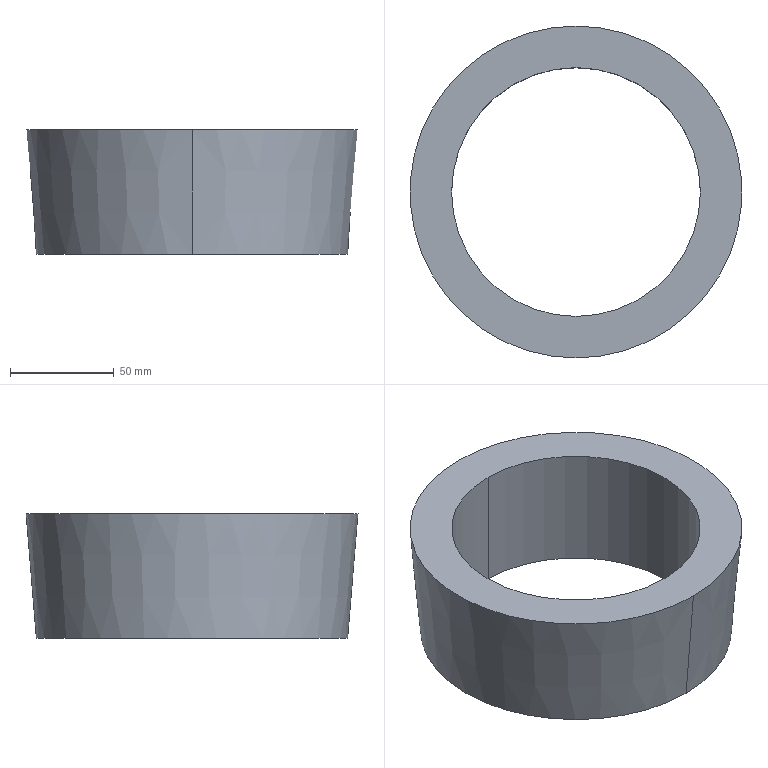Component | SolidWorks | DieCore-1 | 1 solid | 6 faces | box 160.14 x 160.14 x 60 mm | volume 455986 mm3 | cylinder 2 | cone 2 | plane 2 | commonest cylinder face diameters 120 x2
STEP:
#1=CARTESIAN_POINT('',(0.,-2.362,-1.89));
#2=VERTEX_POINT('',#1);
#3=CARTESIAN_POINT('',(-0.,2.362,-1.89));
#4=VERTEX_POINT('',#3);
#5=CARTESIAN_POINT('',(0.,-0.,-1.89));
#6=DIRECTION('',(-0.,0.,-1.));
#7=DIRECTION('',(0.,-1.,-0.));
#8=AXIS2_PLACEMENT_3D('',#5,#6,#7);
#9=CIRCLE('',#8,2.362);
#10=EDGE_CURVE('',#2,#4,#9,.T.);
#11=ORIENTED_EDGE('',*,*,#10,.F.);
#12=CARTESIAN_POINT('',(0.,-2.362,-4.252));
#13=VERTEX_POINT('',#12);
#14=CARTESIAN_POINT('',(0.,-2.362,3.94));
#15=DIRECTION('',(-0.,0.,-1.));
#16=VECTOR('',#15,39.37);
#17=LINE('',#14,#16);
#18=EDGE_CURVE('',#2,#13,#17,.T.);
#19=ORIENTED_EDGE('',*,*,#18,.T.);
#20=CARTESIAN_POINT('',(-0.,2.362,-4.252));
#21=VERTEX_POINT('',#20);
#22=CARTESIAN_POINT('',(0.,-0.,-4.252));
#23=DIRECTION('',(-0.,0.,-1.));
#24=DIRECTION('',(-0.,1.,0.));
#25=AXIS2_PLACEMENT_3D('',#22,#23,#24);
#26=CIRCLE('',#25,2.362);
#27=EDGE_CURVE('',#13,#21,#26,.T.);
#28=ORIENTED_EDGE('',*,*,#27,.T.);
#29=CARTESIAN_POINT('',(0.,2.362,3.94));
#30=DIRECTION('',(-0.,0.,-1.));
#31=VECTOR('',#30,39.37);
#32=LINE('',#29,#31);
#33=EDGE_CURVE('',#4,#21,#32,.T.);
#34=ORIENTED_EDGE('',*,*,#33,.F.);
#35=EDGE_LOOP('',(#11,#19,#28,#34));
#36=FACE_OUTER_BOUND('',#35,.T.);
#37=CARTESIAN_POINT('',(0.,-0.,3.94));
#38=DIRECTION('',(-0.,0.,-1.));
#39=DIRECTION('',(-0.,1.,0.));
#40=AXIS2_PLACEMENT_3D('',#37,#38,#39);
#41=CYLINDRICAL_SURFACE('',#40,2.362);
#42=ADVANCED_FACE('',(#36),#41,.F.);
#43=CARTESIAN_POINT('',(0.,2.955,-4.252));
#44=VERTEX_POINT('',#43);
#45=CARTESIAN_POINT('',(0.,-2.955,-4.252));
#46=VERTEX_POINT('',#45);
#47=CARTESIAN_POINT('',(0.,-0.,-4.252));
#48=DIRECTION('',(-0.,0.,-1.));
#49=DIRECTION('',(-0.,1.,0.));
#50=AXIS2_PLACEMENT_3D('',#47,#48,#49);
#51=CIRCLE('',#50,2.955);
#52=EDGE_CURVE('',#44,#46,#51,.T.);
#53=ORIENTED_EDGE('',*,*,#52,.F.);
#54=CARTESIAN_POINT('',(0.,3.152,-1.89));
#55=VERTEX_POINT('',#54);
#56=CARTESIAN_POINT('',(-0.,2.95,-4.317));
#57=DIRECTION('',(0.,0.08305,0.9965));
#58=VECTOR('',#57,39.37);
#59=LINE('',#56,#58);
#60=EDGE_CURVE('',#44,#55,#59,.T.);
#61=ORIENTED_EDGE('',*,*,#60,.T.);
#62=CARTESIAN_POINT('',(0.,-3.152,-1.89));
#63=VERTEX_POINT('',#62);
#64=CARTESIAN_POINT('',(0.,-0.,-1.89));
#65=DIRECTION('',(-0.,0.,-1.));
#66=DIRECTION('',(0.,-1.,-0.));
#67=AXIS2_PLACEMENT_3D('',#64,#65,#66);
#68=CIRCLE('',#67,3.152);
#69=EDGE_CURVE('',#55,#63,#68,.T.);
#70=ORIENTED_EDGE('',*,*,#69,.T.);
#71=CARTESIAN_POINT('',(0.,-2.95,-4.317));
#72=DIRECTION('',(0.,-0.08305,0.9965));
#73=VECTOR('',#72,39.37);
#74=LINE('',#71,#73);
#75=EDGE_CURVE('',#46,#63,#74,.T.);
#76=ORIENTED_EDGE('',*,*,#75,.F.);
#77=EDGE_LOOP('',(#53,#61,#70,#76));
#78=FACE_OUTER_BOUND('',#77,.T.);
#79=CARTESIAN_POINT('',(0.,-0.,-4.317));
#80=DIRECTION('',(0.,-0.,1.));
#81=DIRECTION('',(0.,-1.,-0.));
#82=AXIS2_PLACEMENT_3D('',#79,#80,#81);
#83=CONICAL_SURFACE('',#82,2.95,0.08314);
#84=ADVANCED_FACE('',(#78),#83,.T.);
#85=CARTESIAN_POINT('',(0.,-0.,-1.89));
#86=DIRECTION('',(-0.,0.,-1.));
#87=DIRECTION('',(0.,-1.,-0.));
#88=AXIS2_PLACEMENT_3D('',#85,#86,#87);
#89=CIRCLE('',#88,3.152);
#90=EDGE_CURVE('',#63,#55,#89,.T.);
#91=ORIENTED_EDGE('',*,*,#90,.F.);
#92=ORIENTED_EDGE('',*,*,#69,.F.);
#93=EDGE_LOOP('',(#91,#92));
#94=FACE_OUTER_BOUND('',#93,.T.);
#95=CARTESIAN_POINT('',(0.,-0.,-1.89));
#96=DIRECTION('',(-0.,0.,-1.));
#97=DIRECTION('',(0.,-1.,-0.));
#98=AXIS2_PLACEMENT_3D('',#95,#96,#97);
#99=CIRCLE('',#98,2.362);
#100=EDGE_CURVE('',#4,#2,#99,.T.);
#101=ORIENTED_EDGE('',*,*,#100,.T.);
#102=ORIENTED_EDGE('',*,*,#10,.T.);
#103=EDGE_LOOP('',(#101,#102));
#104=FACE_BOUND('',#103,.T.);
#105=CARTESIAN_POINT('',(0.,-0.,-1.89));
#106=DIRECTION('',(0.,-0.,1.));
#107=DIRECTION('',(0.,-1.,-0.));
#108=AXIS2_PLACEMENT_3D('',#105,#106,#107);
#109=PLANE('',#108);
#110=ADVANCED_FACE('',(#94,#104),#109,.T.);
#111=ORIENTED_EDGE('',*,*,#60,.F.);
#112=CARTESIAN_POINT('',(0.,-0.,-4.252));
#113=DIRECTION('',(-0.,0.,-1.));
#114=DIRECTION('',(-0.,1.,0.));
#115=AXIS2_PLACEMENT_3D('',#112,#113,#114);
#116=CIRCLE('',#115,2.955);
#117=EDGE_CURVE('',#46,#44,#116,.T.);
#118=ORIENTED_EDGE('',*,*,#117,.F.);
#119=ORIENTED_EDGE('',*,*,#75,.T.);
#120=ORIENTED_EDGE('',*,*,#90,.T.);
#121=EDGE_LOOP('',(#111,#118,#119,#120));
#122=FACE_OUTER_BOUND('',#121,.T.);
#123=CARTESIAN_POINT('',(0.,-0.,-4.317));
#124=DIRECTION('',(0.,-0.,1.));
#125=DIRECTION('',(0.,-1.,-0.));
#126=AXIS2_PLACEMENT_3D('',#123,#124,#125);
#127=CONICAL_SURFACE('',#126,2.95,0.08314);
#128=ADVANCED_FACE('',(#122),#127,.T.);
#129=ORIENTED_EDGE('',*,*,#117,.T.);
#130=ORIENTED_EDGE('',*,*,#52,.T.);
#131=EDGE_LOOP('',(#129,#130));
#132=FACE_OUTER_BOUND('',#131,.T.);
#133=CARTESIAN_POINT('',(0.,-0.,-4.252));
#134=DIRECTION('',(-0.,0.,-1.));
#135=DIRECTION('',(-0.,1.,0.));
#136=AXIS2_PLACEMENT_3D('',#133,#134,#135);
#137=CIRCLE('',#136,2.362);
#138=EDGE_CURVE('',#21,#13,#137,.T.);
#139=ORIENTED_EDGE('',*,*,#138,.F.);
#140=ORIENTED_EDGE('',*,*,#27,.F.);
#141=EDGE_LOOP('',(#139,#140));
#142=FACE_BOUND('',#141,.T.);
#143=CARTESIAN_POINT('',(-0.,2.165,-4.252));
#144=DIRECTION('',(-0.,0.,-1.));
#145=DIRECTION('',(-0.,1.,0.));
#146=AXIS2_PLACEMENT_3D('',#143,#144,#145);
#147=PLANE('',#146);
#148=ADVANCED_FACE('',(#132,#142),#147,.T.);
#149=ORIENTED_EDGE('',*,*,#18,.F.);
#150=ORIENTED_EDGE('',*,*,#100,.F.);
#151=ORIENTED_EDGE('',*,*,#33,.T.);
#152=ORIENTED_EDGE('',*,*,#138,.T.);
#153=EDGE_LOOP('',(#149,#150,#151,#152));
#154=FACE_OUTER_BOUND('',#153,.T.);
#155=CARTESIAN_POINT('',(0.,-0.,3.94));
#156=DIRECTION('',(-0.,0.,-1.));
#157=DIRECTION('',(-0.,1.,0.));
#158=AXIS2_PLACEMENT_3D('',#155,#156,#157);
#159=CYLINDRICAL_SURFACE('',#158,2.362);
#160=ADVANCED_FACE('',(#154),#159,.F.);
#161=CLOSED_SHELL('',(#42,#84,#110,#128,#148,#160));
#162=MANIFOLD_SOLID_BREP('',#161);
#163=CARTESIAN_POINT('',(0.,0.,0.));
#164=DIRECTION('',(0.,0.,1.));
#165=DIRECTION('',(1.,0.,0.));
#166=AXIS2_PLACEMENT_3D('',#163,#164,#165);
#167=(LENGTH_UNIT()NAMED_UNIT(*)SI_UNIT($,.METRE.));
#168=LENGTH_MEASURE_WITH_UNIT(LENGTH_MEASURE(0.0254),#167);
#169=DIMENSIONAL_EXPONENTS(1.,0.,0.,0.,0.,0.,0.);
#170=(CONVERSION_BASED_UNIT('',#168)LENGTH_UNIT()NAMED_UNIT(#169));
#171=UNCERTAINTY_MEASURE_WITH_UNIT(LENGTH_MEASURE(0.00001),#170,'','');
#172=(NAMED_UNIT(*)PLANE_ANGLE_UNIT()SI_UNIT($,.RADIAN.));
#173=(NAMED_UNIT(*)SI_UNIT($,.STERADIAN.)SOLID_ANGLE_UNIT());
#174=(GEOMETRIC_REPRESENTATION_CONTEXT(3)GLOBAL_UNCERTAINTY_ASSIGNED_CONTEXT((#171))GLOBAL_UNIT_ASSIGNED_CONTEXT((#170,#172,#173))REPRESENTATION_CONTEXT('',''));
#175=ADVANCED_BREP_SHAPE_REPRESENTATION('',(#162,#166),#174);
#176=COLOUR_RGB('',0.7922,0.8196,0.9333);
#177=FILL_AREA_STYLE_COLOUR('',#176);
#178=FILL_AREA_STYLE('',(#177));
#179=SURFACE_STYLE_FILL_AREA(#178);
#180=SURFACE_SIDE_STYLE('',(#179));
#181=SURFACE_STYLE_USAGE(.BOTH.,#180);
#182=PRESENTATION_STYLE_ASSIGNMENT((#181));
#183=STYLED_ITEM('',(#182),#162);
#184=(LENGTH_UNIT()NAMED_UNIT(*)SI_UNIT($,.METRE.));
#185=LENGTH_MEASURE_WITH_UNIT(LENGTH_MEASURE(0.0254),#184);
#186=DIMENSIONAL_EXPONENTS(1.,0.,0.,0.,0.,0.,0.);
#187=(CONVERSION_BASED_UNIT('',#185)LENGTH_UNIT()NAMED_UNIT(#186));
#188=UNCERTAINTY_MEASURE_WITH_UNIT(LENGTH_MEASURE(0.00001),#187,'','');
#189=(NAMED_UNIT(*)PLANE_ANGLE_UNIT()SI_UNIT($,.RADIAN.));
#190=(NAMED_UNIT(*)SI_UNIT($,.STERADIAN.)SOLID_ANGLE_UNIT());
#191=(GEOMETRIC_REPRESENTATION_CONTEXT(3)GLOBAL_UNCERTAINTY_ASSIGNED_CONTEXT((#188))GLOBAL_UNIT_ASSIGNED_CONTEXT((#187,#189,#190))REPRESENTATION_CONTEXT('',''));
#192=MECHANICAL_DESIGN_GEOMETRIC_PRESENTATION_REPRESENTATION('',(#183),#191);
#193=PRESENTATION_LAYER_ASSIGNMENT('','',(#183));